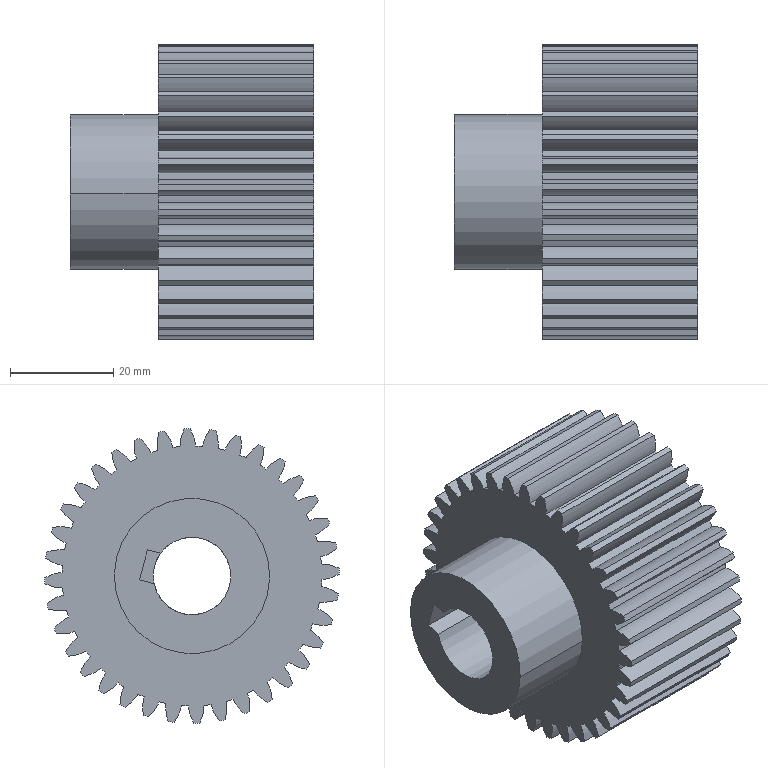Component | SolidWorks | ReducerSmallGear-1 | 1 solid | 155 faces | volume 71476 mm3 | cylinder 76 | spline 72 | plane 7 | commonest cylinder face diameters 50.25 x36 57 x36 30 x2 15 x2